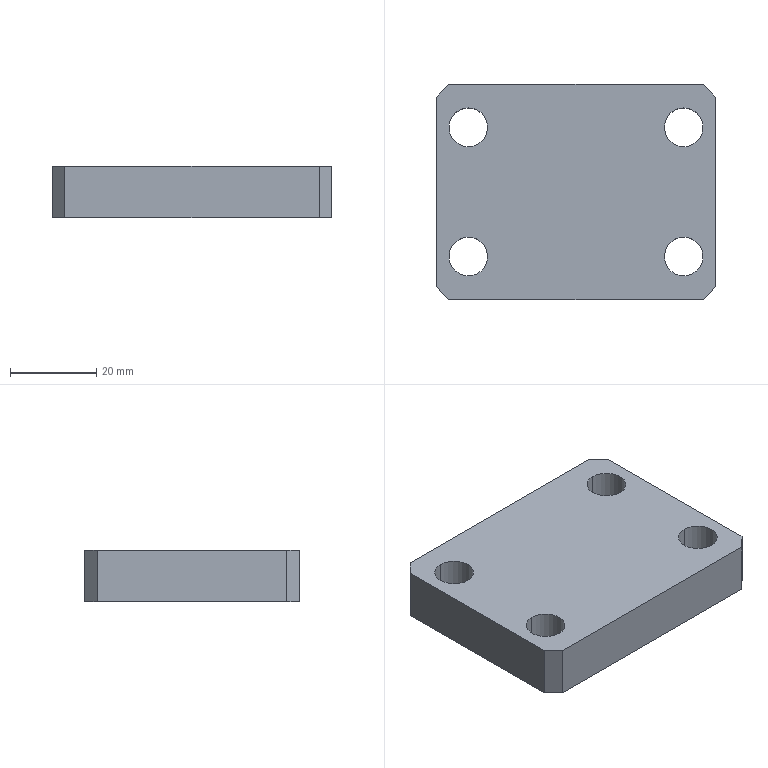Component | SolidWorks | LowerSideBeltXG-XG1-1_LimitTopPlateXG-XG1-1 | 1 solid | 18 faces | box 65 x 50 x 12 mm | volume 35730 mm3 | plane 10 | cylinder 8 | commonest cylinder face diameters 9 x8
build123d program:
from build123d import *

# Parameters (mm, degrees)
SKETCH1_W                = 65
SKETCH1_H                = 50
BOSS_EXTRUDE1_DEPTH      = 6
F_9_0_9_DIAMETER_HOLE1_D = 9
CHAMFER1_SIZE            = 3


with BuildPart() as part:
    # Sketch1 → Boss-Extrude1 (new, symmetric)
    with BuildSketch(Plane(origin=(0, 0, 0), x_dir=(1, 0, 0), z_dir=(0, 1, 0))):
        Rectangle(SKETCH1_W, SKETCH1_H)
    extrude(amount=BOSS_EXTRUDE1_DEPTH, both=True)

    # 9.0 _9_ Diameter Hole1 (through all)
    with Locations(Plane(origin=(0, 6, 0), x_dir=(1, 0, 0), z_dir=(0, 1, 0))):
        with Locations((-25, 15), (-25, -15), (25, 15), (25, -15)):
            Hole(F_9_0_9_DIAMETER_HOLE1_D / 2)

    # Chamfer1
    chamfer1_edges = [part.edges().sort_by_distance(p)[0] for p in [
        (-32.5, 0, -25),
        (32.5, 0, -25),
        (32.5, 0, 25),
        (-32.5, 0, 25),
    ]]
    chamfer(chamfer1_edges, length=CHAMFER1_SIZE)


solid = part.part

# Placed as in the assembly
solid = solid.moved(Location((-348.72, 470, 63), (90, 0, 0)))
STEP:
#1=COLOUR_RGB('',0.7922,0.8196,0.9333);
#2=FILL_AREA_STYLE_COLOUR('',#1);
#3=FILL_AREA_STYLE('',(#2));
#4=SURFACE_STYLE_FILL_AREA(#3);
#5=SURFACE_SIDE_STYLE('',(#4));
#6=SURFACE_STYLE_USAGE(.BOTH.,#5);
#7=PRESENTATION_STYLE_ASSIGNMENT((#6));
#8=CARTESIAN_POINT('',(-14.713,19.272,2.244));
#9=VERTEX_POINT('',#8);
#10=CARTESIAN_POINT('',(-14.713,18.917,2.244));
#11=VERTEX_POINT('',#10);
#12=CARTESIAN_POINT('',(-14.713,19.094,2.244));
#13=DIRECTION('',(0.,-0.,1.));
#14=DIRECTION('',(0.,-1.,0.));
#15=AXIS2_PLACEMENT_3D('',#12,#13,#14);
#16=CIRCLE('',#15,0.1772);
#17=EDGE_CURVE('',#9,#11,#16,.T.);
#18=ORIENTED_EDGE('',*,*,#17,.F.);
#19=CARTESIAN_POINT('',(-14.713,19.272,2.717));
#20=VERTEX_POINT('',#19);
#21=CARTESIAN_POINT('',(-14.713,19.272,2.717));
#22=DIRECTION('',(0.,-0.,1.));
#23=VECTOR('',#22,39.37);
#24=LINE('',#21,#23);
#25=EDGE_CURVE('',#9,#20,#24,.T.);
#26=ORIENTED_EDGE('',*,*,#25,.T.);
#27=CARTESIAN_POINT('',(-14.713,18.917,2.717));
#28=VERTEX_POINT('',#27);
#29=CARTESIAN_POINT('',(-14.713,19.094,2.717));
#30=DIRECTION('',(0.,-0.,1.));
#31=DIRECTION('',(0.,-1.,0.));
#32=AXIS2_PLACEMENT_3D('',#29,#30,#31);
#33=CIRCLE('',#32,0.1772);
#34=EDGE_CURVE('',#20,#28,#33,.T.);
#35=ORIENTED_EDGE('',*,*,#34,.T.);
#36=CARTESIAN_POINT('',(-14.713,18.917,2.717));
#37=DIRECTION('',(0.,-0.,1.));
#38=VECTOR('',#37,39.37);
#39=LINE('',#36,#38);
#40=EDGE_CURVE('',#11,#28,#39,.T.);
#41=ORIENTED_EDGE('',*,*,#40,.F.);
#42=EDGE_LOOP('',(#18,#26,#35,#41));
#43=FACE_OUTER_BOUND('',#42,.T.);
#44=CARTESIAN_POINT('',(-14.713,19.094,2.717));
#45=DIRECTION('',(0.,-0.,1.));
#46=DIRECTION('',(0.,-1.,0.));
#47=AXIS2_PLACEMENT_3D('',#44,#45,#46);
#48=CYLINDRICAL_SURFACE('',#47,0.1772);
#49=ADVANCED_FACE('',(#43),#48,.F.);
#50=CARTESIAN_POINT('',(-14.713,18.091,2.244));
#51=VERTEX_POINT('',#50);
#52=CARTESIAN_POINT('',(-14.713,17.736,2.244));
#53=VERTEX_POINT('',#52);
#54=CARTESIAN_POINT('',(-14.713,17.913,2.244));
#55=DIRECTION('',(0.,-0.,1.));
#56=DIRECTION('',(0.,-1.,0.));
#57=AXIS2_PLACEMENT_3D('',#54,#55,#56);
#58=CIRCLE('',#57,0.1772);
#59=EDGE_CURVE('',#51,#53,#58,.T.);
#60=ORIENTED_EDGE('',*,*,#59,.F.);
#61=CARTESIAN_POINT('',(-14.713,18.091,2.717));
#62=VERTEX_POINT('',#61);
#63=CARTESIAN_POINT('',(-14.713,18.091,2.717));
#64=DIRECTION('',(0.,-0.,1.));
#65=VECTOR('',#64,39.37);
#66=LINE('',#63,#65);
#67=EDGE_CURVE('',#51,#62,#66,.T.);
#68=ORIENTED_EDGE('',*,*,#67,.T.);
#69=CARTESIAN_POINT('',(-14.713,17.736,2.717));
#70=VERTEX_POINT('',#69);
#71=CARTESIAN_POINT('',(-14.713,17.913,2.717));
#72=DIRECTION('',(0.,-0.,1.));
#73=DIRECTION('',(0.,-1.,0.));
#74=AXIS2_PLACEMENT_3D('',#71,#72,#73);
#75=CIRCLE('',#74,0.1772);
#76=EDGE_CURVE('',#62,#70,#75,.T.);
#77=ORIENTED_EDGE('',*,*,#76,.T.);
#78=CARTESIAN_POINT('',(-14.713,17.736,2.717));
#79=DIRECTION('',(0.,-0.,1.));
#80=VECTOR('',#79,39.37);
#81=LINE('',#78,#80);
#82=EDGE_CURVE('',#53,#70,#81,.T.);
#83=ORIENTED_EDGE('',*,*,#82,.F.);
#84=EDGE_LOOP('',(#60,#68,#77,#83));
#85=FACE_OUTER_BOUND('',#84,.T.);
#86=CARTESIAN_POINT('',(-14.713,17.913,2.717));
#87=DIRECTION('',(0.,-0.,1.));
#88=DIRECTION('',(0.,-1.,0.));
#89=AXIS2_PLACEMENT_3D('',#86,#87,#88);
#90=CYLINDRICAL_SURFACE('',#89,0.1772);
#91=ADVANCED_FACE('',(#85),#90,.F.);
#92=CARTESIAN_POINT('',(-12.745,19.272,2.244));
#93=VERTEX_POINT('',#92);
#94=CARTESIAN_POINT('',(-12.745,18.917,2.244));
#95=VERTEX_POINT('',#94);
#96=CARTESIAN_POINT('',(-12.745,19.094,2.244));
#97=DIRECTION('',(0.,-0.,1.));
#98=DIRECTION('',(0.,-1.,0.));
#99=AXIS2_PLACEMENT_3D('',#96,#97,#98);
#100=CIRCLE('',#99,0.1772);
#101=EDGE_CURVE('',#93,#95,#100,.T.);
#102=ORIENTED_EDGE('',*,*,#101,.F.);
#103=CARTESIAN_POINT('',(-12.745,19.272,2.717));
#104=VERTEX_POINT('',#103);
#105=CARTESIAN_POINT('',(-12.745,19.272,2.717));
#106=DIRECTION('',(0.,-0.,1.));
#107=VECTOR('',#106,39.37);
#108=LINE('',#105,#107);
#109=EDGE_CURVE('',#93,#104,#108,.T.);
#110=ORIENTED_EDGE('',*,*,#109,.T.);
#111=CARTESIAN_POINT('',(-12.745,18.917,2.717));
#112=VERTEX_POINT('',#111);
#113=CARTESIAN_POINT('',(-12.745,19.094,2.717));
#114=DIRECTION('',(0.,-0.,1.));
#115=DIRECTION('',(0.,-1.,0.));
#116=AXIS2_PLACEMENT_3D('',#113,#114,#115);
#117=CIRCLE('',#116,0.1772);
#118=EDGE_CURVE('',#104,#112,#117,.T.);
#119=ORIENTED_EDGE('',*,*,#118,.T.);
#120=CARTESIAN_POINT('',(-12.745,18.917,2.717));
#121=DIRECTION('',(0.,-0.,1.));
#122=VECTOR('',#121,39.37);
#123=LINE('',#120,#122);
#124=EDGE_CURVE('',#95,#112,#123,.T.);
#125=ORIENTED_EDGE('',*,*,#124,.F.);
#126=EDGE_LOOP('',(#102,#110,#119,#125));
#127=FACE_OUTER_BOUND('',#126,.T.);
#128=CARTESIAN_POINT('',(-12.745,19.094,2.717));
#129=DIRECTION('',(0.,-0.,1.));
#130=DIRECTION('',(0.,-1.,0.));
#131=AXIS2_PLACEMENT_3D('',#128,#129,#130);
#132=CYLINDRICAL_SURFACE('',#131,0.1772);
#133=ADVANCED_FACE('',(#127),#132,.F.);
#134=CARTESIAN_POINT('',(-12.745,18.091,2.244));
#135=VERTEX_POINT('',#134);
#136=CARTESIAN_POINT('',(-12.745,17.736,2.244));
#137=VERTEX_POINT('',#136);
#138=CARTESIAN_POINT('',(-12.745,17.913,2.244));
#139=DIRECTION('',(0.,-0.,1.));
#140=DIRECTION('',(0.,-1.,0.));
#141=AXIS2_PLACEMENT_3D('',#138,#139,#140);
#142=CIRCLE('',#141,0.1772);
#143=EDGE_CURVE('',#135,#137,#142,.T.);
#144=ORIENTED_EDGE('',*,*,#143,.F.);
#145=CARTESIAN_POINT('',(-12.745,18.091,2.717));
#146=VERTEX_POINT('',#145);
#147=CARTESIAN_POINT('',(-12.745,18.091,2.717));
#148=DIRECTION('',(0.,-0.,1.));
#149=VECTOR('',#148,39.37);
#150=LINE('',#147,#149);
#151=EDGE_CURVE('',#135,#146,#150,.T.);
#152=ORIENTED_EDGE('',*,*,#151,.T.);
#153=CARTESIAN_POINT('',(-12.745,17.736,2.717));
#154=VERTEX_POINT('',#153);
#155=CARTESIAN_POINT('',(-12.745,17.913,2.717));
#156=DIRECTION('',(0.,-0.,1.));
#157=DIRECTION('',(0.,-1.,0.));
#158=AXIS2_PLACEMENT_3D('',#155,#156,#157);
#159=CIRCLE('',#158,0.1772);
#160=EDGE_CURVE('',#146,#154,#159,.T.);
#161=ORIENTED_EDGE('',*,*,#160,.T.);
#162=CARTESIAN_POINT('',(-12.745,17.736,2.717));
#163=DIRECTION('',(0.,-0.,1.));
#164=VECTOR('',#163,39.37);
#165=LINE('',#162,#164);
#166=EDGE_CURVE('',#137,#154,#165,.T.);
#167=ORIENTED_EDGE('',*,*,#166,.F.);
#168=EDGE_LOOP('',(#144,#152,#161,#167));
#169=FACE_OUTER_BOUND('',#168,.T.);
#170=CARTESIAN_POINT('',(-12.745,17.913,2.717));
#171=DIRECTION('',(0.,-0.,1.));
#172=DIRECTION('',(0.,-1.,0.));
#173=AXIS2_PLACEMENT_3D('',#170,#171,#172);
#174=CYLINDRICAL_SURFACE('',#173,0.1772);
#175=ADVANCED_FACE('',(#169),#174,.F.);
#176=CARTESIAN_POINT('',(-15.009,19.37,2.244));
#177=VERTEX_POINT('',#176);
#178=CARTESIAN_POINT('',(-15.009,17.638,2.244));
#179=VERTEX_POINT('',#178);
#180=CARTESIAN_POINT('',(-15.009,17.52,2.244));
#181=DIRECTION('',(0.,-1.,-0.));
#182=VECTOR('',#181,39.37);
#183=LINE('',#180,#182);
#184=EDGE_CURVE('',#177,#179,#183,.T.);
#185=ORIENTED_EDGE('',*,*,#184,.T.);
#186=CARTESIAN_POINT('',(-15.009,17.638,2.717));
#187=VERTEX_POINT('',#186);
#188=CARTESIAN_POINT('',(-15.009,17.638,2.717));
#189=DIRECTION('',(0.,-0.,1.));
#190=VECTOR('',#189,39.37);
#191=LINE('',#188,#190);
#192=EDGE_CURVE('',#179,#187,#191,.T.);
#193=ORIENTED_EDGE('',*,*,#192,.T.);
#194=CARTESIAN_POINT('',(-15.009,19.37,2.717));
#195=VERTEX_POINT('',#194);
#196=CARTESIAN_POINT('',(-15.009,17.52,2.717));
#197=DIRECTION('',(0.,-1.,-0.));
#198=VECTOR('',#197,39.37);
#199=LINE('',#196,#198);
#200=EDGE_CURVE('',#195,#187,#199,.T.);
#201=ORIENTED_EDGE('',*,*,#200,.F.);
#202=CARTESIAN_POINT('',(-15.009,19.37,2.717));
#203=DIRECTION('',(-0.,0.,-1.));
#204=VECTOR('',#203,39.37);
#205=LINE('',#202,#204);
#206=EDGE_CURVE('',#195,#177,#205,.T.);
#207=ORIENTED_EDGE('',*,*,#206,.T.);
#208=EDGE_LOOP('',(#185,#193,#201,#207));
#209=FACE_OUTER_BOUND('',#208,.T.);
#210=CARTESIAN_POINT('',(-15.009,17.52,2.717));
#211=DIRECTION('',(1.,0.,-0.));
#212=DIRECTION('',(-0.,1.,0.));
#213=AXIS2_PLACEMENT_3D('',#210,#211,#212);
#214=PLANE('',#213);
#215=ADVANCED_FACE('',(#209),#214,.F.);
#216=CARTESIAN_POINT('',(-14.891,17.52,2.244));
#217=VERTEX_POINT('',#216);
#218=CARTESIAN_POINT('',(-12.568,17.52,2.244));
#219=VERTEX_POINT('',#218);
#220=CARTESIAN_POINT('',(-12.45,17.52,2.244));
#221=DIRECTION('',(1.,0.,-0.));
#222=VECTOR('',#221,39.37);
#223=LINE('',#220,#222);
#224=EDGE_CURVE('',#217,#219,#223,.T.);
#225=ORIENTED_EDGE('',*,*,#224,.T.);
#226=CARTESIAN_POINT('',(-12.568,17.52,2.717));
#227=VERTEX_POINT('',#226);
#228=CARTESIAN_POINT('',(-12.568,17.52,2.717));
#229=DIRECTION('',(0.,-0.,1.));
#230=VECTOR('',#229,39.37);
#231=LINE('',#228,#230);
#232=EDGE_CURVE('',#219,#227,#231,.T.);
#233=ORIENTED_EDGE('',*,*,#232,.T.);
#234=CARTESIAN_POINT('',(-14.891,17.52,2.717));
#235=VERTEX_POINT('',#234);
#236=CARTESIAN_POINT('',(-12.45,17.52,2.717));
#237=DIRECTION('',(1.,0.,-0.));
#238=VECTOR('',#237,39.37);
#239=LINE('',#236,#238);
#240=EDGE_CURVE('',#235,#227,#239,.T.);
#241=ORIENTED_EDGE('',*,*,#240,.F.);
#242=CARTESIAN_POINT('',(-14.891,17.52,2.717));
#243=DIRECTION('',(-0.,0.,-1.));
#244=VECTOR('',#243,39.37);
#245=LINE('',#242,#244);
#246=EDGE_CURVE('',#235,#217,#245,.T.);
#247=ORIENTED_EDGE('',*,*,#246,.T.);
#248=EDGE_LOOP('',(#225,#233,#241,#247));
#249=FACE_OUTER_BOUND('',#248,.T.);
#250=CARTESIAN_POINT('',(-12.45,17.52,2.717));
#251=DIRECTION('',(-0.,1.,0.));
#252=DIRECTION('',(-1.,-0.,0.));
#253=AXIS2_PLACEMENT_3D('',#250,#251,#252);
#254=PLANE('',#253);
#255=ADVANCED_FACE('',(#249),#254,.F.);
#256=CARTESIAN_POINT('',(-12.45,17.638,2.717));
#257=VERTEX_POINT('',#256);
#258=CARTESIAN_POINT('',(-12.45,19.37,2.717));
#259=VERTEX_POINT('',#258);
#260=CARTESIAN_POINT('',(-12.45,17.52,2.717));
#261=DIRECTION('',(-0.,1.,0.));
#262=VECTOR('',#261,39.37);
#263=LINE('',#260,#262);
#264=EDGE_CURVE('',#257,#259,#263,.T.);
#265=ORIENTED_EDGE('',*,*,#264,.F.);
#266=CARTESIAN_POINT('',(-12.45,17.638,2.244));
#267=VERTEX_POINT('',#266);
#268=CARTESIAN_POINT('',(-12.45,17.638,2.717));
#269=DIRECTION('',(-0.,0.,-1.));
#270=VECTOR('',#269,39.37);
#271=LINE('',#268,#270);
#272=EDGE_CURVE('',#257,#267,#271,.T.);
#273=ORIENTED_EDGE('',*,*,#272,.T.);
#274=CARTESIAN_POINT('',(-12.45,19.37,2.244));
#275=VERTEX_POINT('',#274);
#276=CARTESIAN_POINT('',(-12.45,17.52,2.244));
#277=DIRECTION('',(-0.,1.,0.));
#278=VECTOR('',#277,39.37);
#279=LINE('',#276,#278);
#280=EDGE_CURVE('',#267,#275,#279,.T.);
#281=ORIENTED_EDGE('',*,*,#280,.T.);
#282=CARTESIAN_POINT('',(-12.45,19.37,2.717));
#283=DIRECTION('',(0.,-0.,1.));
#284=VECTOR('',#283,39.37);
#285=LINE('',#282,#284);
#286=EDGE_CURVE('',#275,#259,#285,.T.);
#287=ORIENTED_EDGE('',*,*,#286,.T.);
#288=EDGE_LOOP('',(#265,#273,#281,#287));
#289=FACE_OUTER_BOUND('',#288,.T.);
#290=CARTESIAN_POINT('',(-12.45,17.52,2.717));
#291=DIRECTION('',(-1.,-0.,0.));
#292=DIRECTION('',(0.,-1.,-0.));
#293=AXIS2_PLACEMENT_3D('',#290,#291,#292);
#294=PLANE('',#293);
#295=ADVANCED_FACE('',(#289),#294,.F.);
#296=CARTESIAN_POINT('',(-12.568,19.488,2.244));
#297=VERTEX_POINT('',#296);
#298=CARTESIAN_POINT('',(-14.891,19.488,2.244));
#299=VERTEX_POINT('',#298);
#300=CARTESIAN_POINT('',(-12.45,19.488,2.244));
#301=DIRECTION('',(-1.,-0.,0.));
#302=VECTOR('',#301,39.37);
#303=LINE('',#300,#302);
#304=EDGE_CURVE('',#297,#299,#303,.T.);
#305=ORIENTED_EDGE('',*,*,#304,.T.);
#306=CARTESIAN_POINT('',(-14.891,19.488,2.717));
#307=VERTEX_POINT('',#306);
#308=CARTESIAN_POINT('',(-14.891,19.488,2.717));
#309=DIRECTION('',(0.,-0.,1.));
#310=VECTOR('',#309,39.37);
#311=LINE('',#308,#310);
#312=EDGE_CURVE('',#299,#307,#311,.T.);
#313=ORIENTED_EDGE('',*,*,#312,.T.);
#314=CARTESIAN_POINT('',(-12.568,19.488,2.717));
#315=VERTEX_POINT('',#314);
#316=CARTESIAN_POINT('',(-12.45,19.488,2.717));
#317=DIRECTION('',(-1.,-0.,0.));
#318=VECTOR('',#317,39.37);
#319=LINE('',#316,#318);
#320=EDGE_CURVE('',#315,#307,#319,.T.);
#321=ORIENTED_EDGE('',*,*,#320,.F.);
#322=CARTESIAN_POINT('',(-12.568,19.488,2.717));
#323=DIRECTION('',(-0.,0.,-1.));
#324=VECTOR('',#323,39.37);
#325=LINE('',#322,#324);
#326=EDGE_CURVE('',#315,#297,#325,.T.);
#327=ORIENTED_EDGE('',*,*,#326,.T.);
#328=EDGE_LOOP('',(#305,#313,#321,#327));
#329=FACE_OUTER_BOUND('',#328,.T.);
#330=CARTESIAN_POINT('',(-12.45,19.488,2.717));
#331=DIRECTION('',(0.,-1.,-0.));
#332=DIRECTION('',(1.,0.,-0.));
#333=AXIS2_PLACEMENT_3D('',#330,#331,#332);
#334=PLANE('',#333);
#335=ADVANCED_FACE('',(#329),#334,.F.);
#336=CARTESIAN_POINT('',(-14.713,19.094,2.717));
#337=DIRECTION('',(0.,-0.,1.));
#338=DIRECTION('',(0.,-1.,0.));
#339=AXIS2_PLACEMENT_3D('',#336,#337,#338);
#340=CIRCLE('',#339,0.1772);
#341=EDGE_CURVE('',#28,#20,#340,.T.);
#342=ORIENTED_EDGE('',*,*,#341,.F.);
#343=ORIENTED_EDGE('',*,*,#34,.F.);
#344=EDGE_LOOP('',(#342,#343));
#345=FACE_BOUND('',#344,.T.);
#346=CARTESIAN_POINT('',(-14.713,17.913,2.717));
#347=DIRECTION('',(0.,-0.,1.));
#348=DIRECTION('',(0.,-1.,0.));
#349=AXIS2_PLACEMENT_3D('',#346,#347,#348);
#350=CIRCLE('',#349,0.1772);
#351=EDGE_CURVE('',#70,#62,#350,.T.);
#352=ORIENTED_EDGE('',*,*,#351,.F.);
#353=ORIENTED_EDGE('',*,*,#76,.F.);
#354=EDGE_LOOP('',(#352,#353));
#355=FACE_BOUND('',#354,.T.);
#356=CARTESIAN_POINT('',(-12.745,19.094,2.717));
#357=DIRECTION('',(0.,-0.,1.));
#358=DIRECTION('',(0.,-1.,0.));
#359=AXIS2_PLACEMENT_3D('',#356,#357,#358);
#360=CIRCLE('',#359,0.1772);
#361=EDGE_CURVE('',#112,#104,#360,.T.);
#362=ORIENTED_EDGE('',*,*,#361,.F.);
#363=ORIENTED_EDGE('',*,*,#118,.F.);
#364=EDGE_LOOP('',(#362,#363));
#365=FACE_BOUND('',#364,.T.);
#366=CARTESIAN_POINT('',(-12.745,17.913,2.717));
#367=DIRECTION('',(0.,-0.,1.));
#368=DIRECTION('',(0.,-1.,0.));
#369=AXIS2_PLACEMENT_3D('',#366,#367,#368);
#370=CIRCLE('',#369,0.1772);
#371=EDGE_CURVE('',#154,#146,#370,.T.);
#372=ORIENTED_EDGE('',*,*,#371,.F.);
#373=ORIENTED_EDGE('',*,*,#160,.F.);
#374=EDGE_LOOP('',(#372,#373));
#375=FACE_BOUND('',#374,.T.);
#376=ORIENTED_EDGE('',*,*,#240,.T.);
#377=CARTESIAN_POINT('',(-12.656,17.431,2.717));
#378=DIRECTION('',(0.7071,0.7071,0.));
#379=VECTOR('',#378,39.37);
#380=LINE('',#377,#379);
#381=EDGE_CURVE('',#227,#257,#380,.T.);
#382=ORIENTED_EDGE('',*,*,#381,.T.);
#383=ORIENTED_EDGE('',*,*,#264,.T.);
#384=CARTESIAN_POINT('',(-12.656,19.577,2.717));
#385=DIRECTION('',(-0.7071,0.7071,0.));
#386=VECTOR('',#385,39.37);
#387=LINE('',#384,#386);
#388=EDGE_CURVE('',#259,#315,#387,.T.);
#389=ORIENTED_EDGE('',*,*,#388,.T.);
#390=ORIENTED_EDGE('',*,*,#320,.T.);
#391=CARTESIAN_POINT('',(-14.802,19.577,2.717));
#392=DIRECTION('',(-0.7071,-0.7071,-0.));
#393=VECTOR('',#392,39.37);
#394=LINE('',#391,#393);
#395=EDGE_CURVE('',#307,#195,#394,.T.);
#396=ORIENTED_EDGE('',*,*,#395,.T.);
#397=ORIENTED_EDGE('',*,*,#200,.T.);
#398=CARTESIAN_POINT('',(-14.802,17.431,2.717));
#399=DIRECTION('',(0.7071,-0.7071,-0.));
#400=VECTOR('',#399,39.37);
#401=LINE('',#398,#400);
#402=EDGE_CURVE('',#187,#235,#401,.T.);
#403=ORIENTED_EDGE('',*,*,#402,.T.);
#404=EDGE_LOOP('',(#376,#382,#383,#389,#390,#396,#397,#403));
#405=FACE_OUTER_BOUND('',#404,.T.);
#406=CARTESIAN_POINT('',(-13.729,18.504,2.717));
#407=DIRECTION('',(0.,-0.,1.));
#408=DIRECTION('',(0.,-1.,-0.));
#409=AXIS2_PLACEMENT_3D('',#406,#407,#408);
#410=PLANE('',#409);
#411=ADVANCED_FACE('',(#345,#355,#365,#375,#405),#410,.T.);
#412=CARTESIAN_POINT('',(-14.713,19.094,2.244));
#413=DIRECTION('',(0.,-0.,1.));
#414=DIRECTION('',(0.,-1.,0.));
#415=AXIS2_PLACEMENT_3D('',#412,#413,#414);
#416=CIRCLE('',#415,0.1772);
#417=EDGE_CURVE('',#11,#9,#416,.T.);
#418=ORIENTED_EDGE('',*,*,#417,.T.);
#419=ORIENTED_EDGE('',*,*,#17,.T.);
#420=EDGE_LOOP('',(#418,#419));
#421=FACE_BOUND('',#420,.T.);
#422=CARTESIAN_POINT('',(-14.713,17.913,2.244));
#423=DIRECTION('',(0.,-0.,1.));
#424=DIRECTION('',(0.,-1.,0.));
#425=AXIS2_PLACEMENT_3D('',#422,#423,#424);
#426=CIRCLE('',#425,0.1772);
#427=EDGE_CURVE('',#53,#51,#426,.T.);
#428=ORIENTED_EDGE('',*,*,#427,.T.);
#429=ORIENTED_EDGE('',*,*,#59,.T.);
#430=EDGE_LOOP('',(#428,#429));
#431=FACE_BOUND('',#430,.T.);
#432=CARTESIAN_POINT('',(-12.745,19.094,2.244));
#433=DIRECTION('',(0.,-0.,1.));
#434=DIRECTION('',(0.,-1.,0.));
#435=AXIS2_PLACEMENT_3D('',#432,#433,#434);
#436=CIRCLE('',#435,0.1772);
#437=EDGE_CURVE('',#95,#93,#436,.T.);
#438=ORIENTED_EDGE('',*,*,#437,.T.);
#439=ORIENTED_EDGE('',*,*,#101,.T.);
#440=EDGE_LOOP('',(#438,#439));
#441=FACE_BOUND('',#440,.T.);
#442=CARTESIAN_POINT('',(-12.745,17.913,2.244));
#443=DIRECTION('',(0.,-0.,1.));
#444=DIRECTION('',(0.,-1.,0.));
#445=AXIS2_PLACEMENT_3D('',#442,#443,#444);
#446=CIRCLE('',#445,0.1772);
#447=EDGE_CURVE('',#137,#135,#446,.T.);
#448=ORIENTED_EDGE('',*,*,#447,.T.);
#449=ORIENTED_EDGE('',*,*,#143,.T.);
#450=EDGE_LOOP('',(#448,#449));
#451=FACE_BOUND('',#450,.T.);
#452=ORIENTED_EDGE('',*,*,#280,.F.);
#453=CARTESIAN_POINT('',(-12.45,17.638,2.244));
#454=DIRECTION('',(-0.7071,-0.7071,-0.));
#455=VECTOR('',#454,39.37);
#456=LINE('',#453,#455);
#457=EDGE_CURVE('',#267,#219,#456,.T.);
#458=ORIENTED_EDGE('',*,*,#457,.T.);
#459=ORIENTED_EDGE('',*,*,#224,.F.);
#460=CARTESIAN_POINT('',(-14.891,17.52,2.244));
#461=DIRECTION('',(-0.7071,0.7071,0.));
#462=VECTOR('',#461,39.37);
#463=LINE('',#460,#462);
#464=EDGE_CURVE('',#217,#179,#463,.T.);
#465=ORIENTED_EDGE('',*,*,#464,.T.);
#466=ORIENTED_EDGE('',*,*,#184,.F.);
#467=CARTESIAN_POINT('',(-15.009,19.37,2.244));
#468=DIRECTION('',(0.7071,0.7071,0.));
#469=VECTOR('',#468,39.37);
#470=LINE('',#467,#469);
#471=EDGE_CURVE('',#177,#299,#470,.T.);
#472=ORIENTED_EDGE('',*,*,#471,.T.);
#473=ORIENTED_EDGE('',*,*,#304,.F.);
#474=CARTESIAN_POINT('',(-12.568,19.488,2.244));
#475=DIRECTION('',(0.7071,-0.7071,-0.));
#476=VECTOR('',#475,39.37);
#477=LINE('',#474,#476);
#478=EDGE_CURVE('',#297,#275,#477,.T.);
#479=ORIENTED_EDGE('',*,*,#478,.T.);
#480=EDGE_LOOP('',(#452,#458,#459,#465,#466,#472,#473,#479));
#481=FACE_OUTER_BOUND('',#480,.T.);
#482=CARTESIAN_POINT('',(-13.729,18.504,2.244));
#483=DIRECTION('',(0.,-0.,1.));
#484=DIRECTION('',(0.,-1.,-0.));
#485=AXIS2_PLACEMENT_3D('',#482,#483,#484);
#486=PLANE('',#485);
#487=ADVANCED_FACE('',(#421,#431,#441,#451,#481),#486,.F.);
#488=ORIENTED_EDGE('',*,*,#151,.F.);
#489=ORIENTED_EDGE('',*,*,#447,.F.);
#490=ORIENTED_EDGE('',*,*,#166,.T.);
#491=ORIENTED_EDGE('',*,*,#371,.T.);
#492=EDGE_LOOP('',(#488,#489,#490,#491));
#493=FACE_OUTER_BOUND('',#492,.T.);
#494=CARTESIAN_POINT('',(-12.745,17.913,2.717));
#495=DIRECTION('',(0.,-0.,1.));
#496=DIRECTION('',(0.,-1.,0.));
#497=AXIS2_PLACEMENT_3D('',#494,#495,#496);
#498=CYLINDRICAL_SURFACE('',#497,0.1772);
#499=ADVANCED_FACE('',(#493),#498,.F.);
#500=ORIENTED_EDGE('',*,*,#109,.F.);
#501=ORIENTED_EDGE('',*,*,#437,.F.);
#502=ORIENTED_EDGE('',*,*,#124,.T.);
#503=ORIENTED_EDGE('',*,*,#361,.T.);
#504=EDGE_LOOP('',(#500,#501,#502,#503));
#505=FACE_OUTER_BOUND('',#504,.T.);
#506=CARTESIAN_POINT('',(-12.745,19.094,2.717));
#507=DIRECTION('',(0.,-0.,1.));
#508=DIRECTION('',(0.,-1.,0.));
#509=AXIS2_PLACEMENT_3D('',#506,#507,#508);
#510=CYLINDRICAL_SURFACE('',#509,0.1772);
#511=ADVANCED_FACE('',(#505),#510,.F.);
#512=ORIENTED_EDGE('',*,*,#67,.F.);
#513=ORIENTED_EDGE('',*,*,#427,.F.);
#514=ORIENTED_EDGE('',*,*,#82,.T.);
#515=ORIENTED_EDGE('',*,*,#351,.T.);
#516=EDGE_LOOP('',(#512,#513,#514,#515));
#517=FACE_OUTER_BOUND('',#516,.T.);
#518=CARTESIAN_POINT('',(-14.713,17.913,2.717));
#519=DIRECTION('',(0.,-0.,1.));
#520=DIRECTION('',(0.,-1.,0.));
#521=AXIS2_PLACEMENT_3D('',#518,#519,#520);
#522=CYLINDRICAL_SURFACE('',#521,0.1772);
#523=ADVANCED_FACE('',(#517),#522,.F.);
#524=ORIENTED_EDGE('',*,*,#25,.F.);
#525=ORIENTED_EDGE('',*,*,#417,.F.);
#526=ORIENTED_EDGE('',*,*,#40,.T.);
#527=ORIENTED_EDGE('',*,*,#341,.T.);
#528=EDGE_LOOP('',(#524,#525,#526,#527));
#529=FACE_OUTER_BOUND('',#528,.T.);
#530=CARTESIAN_POINT('',(-14.713,19.094,2.717));
#531=DIRECTION('',(0.,-0.,1.));
#532=DIRECTION('',(0.,-1.,0.));
#533=AXIS2_PLACEMENT_3D('',#530,#531,#532);
#534=CYLINDRICAL_SURFACE('',#533,0.1772);
#535=ADVANCED_FACE('',(#529),#534,.F.);
#536=ORIENTED_EDGE('',*,*,#381,.F.);
#537=ORIENTED_EDGE('',*,*,#232,.F.);
#538=ORIENTED_EDGE('',*,*,#457,.F.);
#539=ORIENTED_EDGE('',*,*,#272,.F.);
#540=EDGE_LOOP('',(#536,#537,#538,#539));
#541=FACE_OUTER_BOUND('',#540,.T.);
#542=CARTESIAN_POINT('',(-12.45,17.638,2.717));
#543=DIRECTION('',(-0.7071,0.7071,0.));
#544=DIRECTION('',(-0.,0.,-1.));
#545=AXIS2_PLACEMENT_3D('',#542,#543,#544);
#546=PLANE('',#545);
#547=ADVANCED_FACE('',(#541),#546,.F.);
#548=ORIENTED_EDGE('',*,*,#402,.F.);
#549=ORIENTED_EDGE('',*,*,#192,.F.);
#550=ORIENTED_EDGE('',*,*,#464,.F.);
#551=ORIENTED_EDGE('',*,*,#246,.F.);
#552=EDGE_LOOP('',(#548,#549,#550,#551));
#553=FACE_OUTER_BOUND('',#552,.T.);
#554=CARTESIAN_POINT('',(-14.891,17.52,2.717));
#555=DIRECTION('',(0.7071,0.7071,0.));
#556=DIRECTION('',(-0.,0.,-1.));
#557=AXIS2_PLACEMENT_3D('',#554,#555,#556);
#558=PLANE('',#557);
#559=ADVANCED_FACE('',(#553),#558,.F.);
#560=ORIENTED_EDGE('',*,*,#395,.F.);
#561=ORIENTED_EDGE('',*,*,#312,.F.);
#562=ORIENTED_EDGE('',*,*,#471,.F.);
#563=ORIENTED_EDGE('',*,*,#206,.F.);
#564=EDGE_LOOP('',(#560,#561,#562,#563));
#565=FACE_OUTER_BOUND('',#564,.T.);
#566=CARTESIAN_POINT('',(-15.009,19.37,2.717));
#567=DIRECTION('',(0.7071,-0.7071,-0.));
#568=DIRECTION('',(-0.,0.,-1.));
#569=AXIS2_PLACEMENT_3D('',#566,#567,#568);
#570=PLANE('',#569);
#571=ADVANCED_FACE('',(#565),#570,.F.);
#572=ORIENTED_EDGE('',*,*,#388,.F.);
#573=ORIENTED_EDGE('',*,*,#286,.F.);
#574=ORIENTED_EDGE('',*,*,#478,.F.);
#575=ORIENTED_EDGE('',*,*,#326,.F.);
#576=EDGE_LOOP('',(#572,#573,#574,#575));
#577=FACE_OUTER_BOUND('',#576,.T.);
#578=CARTESIAN_POINT('',(-12.568,19.488,2.717));
#579=DIRECTION('',(-0.7071,-0.7071,-0.));
#580=DIRECTION('',(-0.,0.,-1.));
#581=AXIS2_PLACEMENT_3D('',#578,#579,#580);
#582=PLANE('',#581);
#583=ADVANCED_FACE('',(#577),#582,.F.);
#584=CLOSED_SHELL('',(#49,#91,#133,#175,#215,#255,#295,#335,#411,#487,#499,#511,#523,#535,#547,#559,#571,#583));
#585=MANIFOLD_SOLID_BREP('',#584);
#586=STYLED_ITEM('',(#7),#585);
#587=PRESENTATION_LAYER_ASSIGNMENT('','',(#586));
#588=(LENGTH_UNIT()NAMED_UNIT(*)SI_UNIT($,.METRE.));
#589=LENGTH_MEASURE_WITH_UNIT(LENGTH_MEASURE(0.0254),#588);
#590=DIMENSIONAL_EXPONENTS(1.,0.,0.,0.,0.,0.,0.);
#591=(CONVERSION_BASED_UNIT('',#589)LENGTH_UNIT()NAMED_UNIT(#590));
#592=UNCERTAINTY_MEASURE_WITH_UNIT(LENGTH_MEASURE(0.00001),#591,'','');
#593=(NAMED_UNIT(*)PLANE_ANGLE_UNIT()SI_UNIT($,.RADIAN.));
#594=(NAMED_UNIT(*)SI_UNIT($,.STERADIAN.)SOLID_ANGLE_UNIT());
#595=(GEOMETRIC_REPRESENTATION_CONTEXT(3)GLOBAL_UNCERTAINTY_ASSIGNED_CONTEXT((#592))GLOBAL_UNIT_ASSIGNED_CONTEXT((#591,#593,#594))REPRESENTATION_CONTEXT('',''));
#596=MECHANICAL_DESIGN_GEOMETRIC_PRESENTATION_REPRESENTATION('',(#586),#595);
#597=CARTESIAN_POINT('',(0.,0.,0.));
#598=DIRECTION('',(0.,0.,1.));
#599=DIRECTION('',(1.,0.,0.));
#600=AXIS2_PLACEMENT_3D('',#597,#598,#599);
#601=(LENGTH_UNIT()NAMED_UNIT(*)SI_UNIT($,.METRE.));
#602=LENGTH_MEASURE_WITH_UNIT(LENGTH_MEASURE(0.0254),#601);
#603=DIMENSIONAL_EXPONENTS(1.,0.,0.,0.,0.,0.,0.);
#604=(CONVERSION_BASED_UNIT('',#602)LENGTH_UNIT()NAMED_UNIT(#603));
#605=UNCERTAINTY_MEASURE_WITH_UNIT(LENGTH_MEASURE(0.00001),#604,'','');
#606=(NAMED_UNIT(*)PLANE_ANGLE_UNIT()SI_UNIT($,.RADIAN.));
#607=(NAMED_UNIT(*)SI_UNIT($,.STERADIAN.)SOLID_ANGLE_UNIT());
#608=(GEOMETRIC_REPRESENTATION_CONTEXT(3)GLOBAL_UNCERTAINTY_ASSIGNED_CONTEXT((#605))GLOBAL_UNIT_ASSIGNED_CONTEXT((#604,#606,#607))REPRESENTATION_CONTEXT('',''));
#609=ADVANCED_BREP_SHAPE_REPRESENTATION('',(#585,#600),#608);